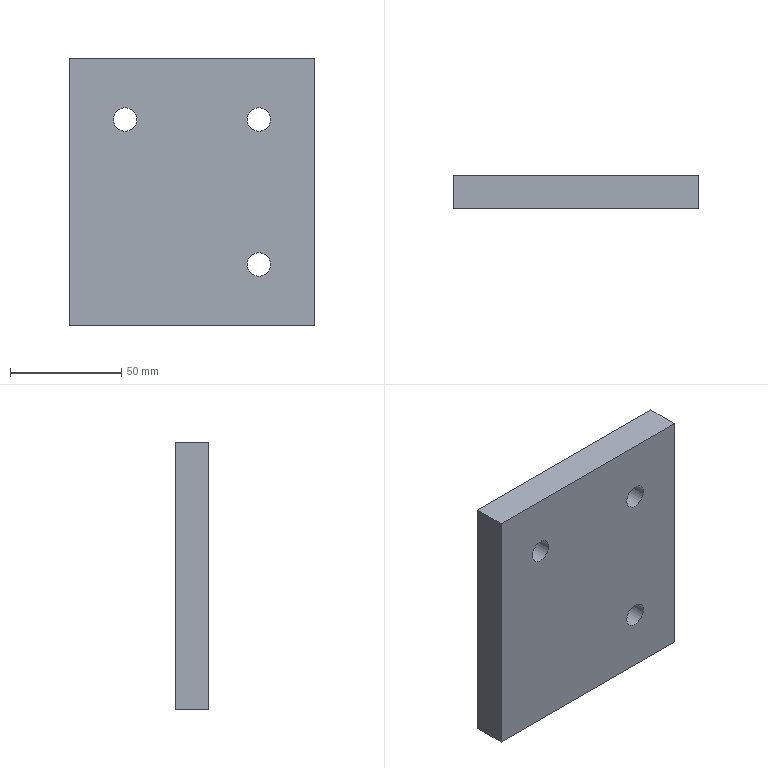Component | NX | FIXED_PLATE_2 | 1 solid | 9 faces | box 110 x 15 x 120 mm | volume 194103 mm3 | plane 6 | cylinder 3 | commonest cylinder face diameters 10.5 x3
STEP:
#1=CARTESIAN_POINT('',(0.,0.,0.));
#2=DIRECTION('',(0.,0.,1.));
#3=DIRECTION('',(1.,0.,0.));
#4=AXIS2_PLACEMENT_3D('',#1,#2,#3);
#5=CARTESIAN_POINT('',(1379.254,1145.,643.5));
#6=VERTEX_POINT('',#5);
#7=CARTESIAN_POINT('',(1379.254,1145.,763.5));
#8=VERTEX_POINT('',#7);
#9=CARTESIAN_POINT('',(1379.254,1145.,643.5));
#10=DIRECTION('',(0.,0.,1.));
#11=VECTOR('',#10,1.);
#12=LINE('',#9,#11);
#13=CARTESIAN_POINT('',(1379.254,1160.,643.5));
#14=DIRECTION('',(1.,0.,0.));
#15=DIRECTION('',(0.,0.,-1.));
#16=AXIS2_PLACEMENT_3D('',#13,#14,#15);
#17=PLANE('',#16);
#18=CARTESIAN_POINT('',(0.,-15.));
#19=DIRECTION('',(-1.,0.));
#20=VECTOR('',#19,1.);
#21=LINE('',#18,#20);
#22=(GEOMETRIC_REPRESENTATION_CONTEXT(2)PARAMETRIC_REPRESENTATION_CONTEXT()REPRESENTATION_CONTEXT('',''));
#23=DEFINITIONAL_REPRESENTATION('',(#21),#22);
#24=PCURVE('',#17,#23);
#25=CARTESIAN_POINT('',(1404.254,1145.,736.));
#26=DIRECTION('',(0.,1.,0.));
#27=DIRECTION('',(0.,0.,1.));
#28=AXIS2_PLACEMENT_3D('',#25,#26,#27);
#29=PLANE('',#28);
#30=CARTESIAN_POINT('',(-92.5,-25.));
#31=DIRECTION('',(1.,0.));
#32=VECTOR('',#31,1.);
#33=LINE('',#30,#32);
#34=(GEOMETRIC_REPRESENTATION_CONTEXT(2)PARAMETRIC_REPRESENTATION_CONTEXT()REPRESENTATION_CONTEXT('',''));
#35=DEFINITIONAL_REPRESENTATION('',(#33),#34);
#36=PCURVE('',#29,#35);
#37=SURFACE_CURVE('',#12,(#24,#36),.PCURVE_S1.);
#38=EDGE_CURVE('',#6,#8,#37,.T.);
#39=ORIENTED_EDGE('',*,*,#38,.T.);
#40=CARTESIAN_POINT('',(1379.254,1160.,763.5));
#41=VERTEX_POINT('',#40);
#42=CARTESIAN_POINT('',(1379.254,1160.,763.5));
#43=DIRECTION('',(0.,-1.,0.));
#44=VECTOR('',#43,1.);
#45=LINE('',#42,#44);
#46=CARTESIAN_POINT('',(-120.,0.));
#47=DIRECTION('',(0.,-1.));
#48=VECTOR('',#47,1.);
#49=LINE('',#46,#48);
#50=(GEOMETRIC_REPRESENTATION_CONTEXT(2)PARAMETRIC_REPRESENTATION_CONTEXT()REPRESENTATION_CONTEXT('',''));
#51=DEFINITIONAL_REPRESENTATION('',(#49),#50);
#52=PCURVE('',#17,#51);
#53=CARTESIAN_POINT('',(1379.254,1160.,763.5));
#54=DIRECTION('',(0.,0.,-1.));
#55=DIRECTION('',(-1.,0.,-0.));
#56=AXIS2_PLACEMENT_3D('',#53,#54,#55);
#57=PLANE('',#56);
#58=CARTESIAN_POINT('',(0.,0.));
#59=DIRECTION('',(0.,-1.));
#60=VECTOR('',#59,1.);
#61=LINE('',#58,#60);
#62=(GEOMETRIC_REPRESENTATION_CONTEXT(2)PARAMETRIC_REPRESENTATION_CONTEXT()REPRESENTATION_CONTEXT('',''));
#63=DEFINITIONAL_REPRESENTATION('',(#61),#62);
#64=PCURVE('',#57,#63);
#65=SURFACE_CURVE('',#45,(#52,#64),.PCURVE_S1.);
#66=EDGE_CURVE('',#41,#8,#65,.T.);
#67=ORIENTED_EDGE('',*,*,#66,.F.);
#68=CARTESIAN_POINT('',(1379.254,1160.,643.5));
#69=VERTEX_POINT('',#68);
#70=CARTESIAN_POINT('',(1379.254,1160.,643.5));
#71=DIRECTION('',(0.,0.,1.));
#72=VECTOR('',#71,1.);
#73=LINE('',#70,#72);
#74=CARTESIAN_POINT('',(0.,0.));
#75=DIRECTION('',(-1.,0.));
#76=VECTOR('',#75,1.);
#77=LINE('',#74,#76);
#78=(GEOMETRIC_REPRESENTATION_CONTEXT(2)PARAMETRIC_REPRESENTATION_CONTEXT()REPRESENTATION_CONTEXT('',''));
#79=DEFINITIONAL_REPRESENTATION('',(#77),#78);
#80=PCURVE('',#17,#79);
#81=CARTESIAN_POINT('',(1404.254,1160.,736.));
#82=DIRECTION('',(0.,1.,0.));
#83=DIRECTION('',(0.,0.,1.));
#84=AXIS2_PLACEMENT_3D('',#81,#82,#83);
#85=PLANE('',#84);
#86=CARTESIAN_POINT('',(-92.5,-25.));
#87=DIRECTION('',(1.,0.));
#88=VECTOR('',#87,1.);
#89=LINE('',#86,#88);
#90=(GEOMETRIC_REPRESENTATION_CONTEXT(2)PARAMETRIC_REPRESENTATION_CONTEXT()REPRESENTATION_CONTEXT('',''));
#91=DEFINITIONAL_REPRESENTATION('',(#89),#90);
#92=PCURVE('',#85,#91);
#93=SURFACE_CURVE('',#73,(#80,#92),.PCURVE_S1.);
#94=EDGE_CURVE('',#69,#41,#93,.T.);
#95=ORIENTED_EDGE('',*,*,#94,.F.);
#96=CARTESIAN_POINT('',(1379.254,1160.,643.5));
#97=DIRECTION('',(0.,-1.,0.));
#98=VECTOR('',#97,1.);
#99=LINE('',#96,#98);
#100=CARTESIAN_POINT('',(0.,0.));
#101=DIRECTION('',(0.,-1.));
#102=VECTOR('',#101,1.);
#103=LINE('',#100,#102);
#104=(GEOMETRIC_REPRESENTATION_CONTEXT(2)PARAMETRIC_REPRESENTATION_CONTEXT()REPRESENTATION_CONTEXT('',''));
#105=DEFINITIONAL_REPRESENTATION('',(#103),#104);
#106=PCURVE('',#17,#105);
#107=CARTESIAN_POINT('',(1489.254,1160.,643.5));
#108=DIRECTION('',(0.,0.,1.));
#109=DIRECTION('',(1.,0.,0.));
#110=AXIS2_PLACEMENT_3D('',#107,#108,#109);
#111=PLANE('',#110);
#112=CARTESIAN_POINT('',(-110.,0.));
#113=DIRECTION('',(0.,-1.));
#114=VECTOR('',#113,1.);
#115=LINE('',#112,#114);
#116=(GEOMETRIC_REPRESENTATION_CONTEXT(2)PARAMETRIC_REPRESENTATION_CONTEXT()REPRESENTATION_CONTEXT('',''));
#117=DEFINITIONAL_REPRESENTATION('',(#115),#116);
#118=PCURVE('',#111,#117);
#119=SURFACE_CURVE('',#99,(#106,#118),.PCURVE_S1.);
#120=EDGE_CURVE('',#69,#6,#119,.T.);
#121=ORIENTED_EDGE('',*,*,#120,.T.);
#122=EDGE_LOOP('',(#39,#67,#95,#121));
#123=FACE_BOUND('',#122,.T.);
#124=ADVANCED_FACE('',(#123),#17,.F.);
#125=CARTESIAN_POINT('',(1489.254,1145.,763.5));
#126=VERTEX_POINT('',#125);
#127=CARTESIAN_POINT('',(1379.254,1145.,763.5));
#128=DIRECTION('',(1.,0.,0.));
#129=VECTOR('',#128,1.);
#130=LINE('',#127,#129);
#131=CARTESIAN_POINT('',(0.,-15.));
#132=DIRECTION('',(-1.,0.));
#133=VECTOR('',#132,1.);
#134=LINE('',#131,#133);
#135=(GEOMETRIC_REPRESENTATION_CONTEXT(2)PARAMETRIC_REPRESENTATION_CONTEXT()REPRESENTATION_CONTEXT('',''));
#136=DEFINITIONAL_REPRESENTATION('',(#134),#135);
#137=PCURVE('',#57,#136);
#138=CARTESIAN_POINT('',(27.5,-25.));
#139=DIRECTION('',(0.,1.));
#140=VECTOR('',#139,1.);
#141=LINE('',#138,#140);
#142=(GEOMETRIC_REPRESENTATION_CONTEXT(2)PARAMETRIC_REPRESENTATION_CONTEXT()REPRESENTATION_CONTEXT('',''));
#143=DEFINITIONAL_REPRESENTATION('',(#141),#142);
#144=PCURVE('',#29,#143);
#145=SURFACE_CURVE('',#130,(#137,#144),.PCURVE_S1.);
#146=EDGE_CURVE('',#8,#126,#145,.T.);
#147=ORIENTED_EDGE('',*,*,#146,.T.);
#148=CARTESIAN_POINT('',(1489.254,1160.,763.5));
#149=VERTEX_POINT('',#148);
#150=CARTESIAN_POINT('',(1489.254,1160.,763.5));
#151=DIRECTION('',(0.,-1.,0.));
#152=VECTOR('',#151,1.);
#153=LINE('',#150,#152);
#154=CARTESIAN_POINT('',(-110.,0.));
#155=DIRECTION('',(0.,-1.));
#156=VECTOR('',#155,1.);
#157=LINE('',#154,#156);
#158=(GEOMETRIC_REPRESENTATION_CONTEXT(2)PARAMETRIC_REPRESENTATION_CONTEXT()REPRESENTATION_CONTEXT('',''));
#159=DEFINITIONAL_REPRESENTATION('',(#157),#158);
#160=PCURVE('',#57,#159);
#161=CARTESIAN_POINT('',(1489.254,1160.,763.5));
#162=DIRECTION('',(-1.,0.,-0.));
#163=DIRECTION('',(-0.,0.,1.));
#164=AXIS2_PLACEMENT_3D('',#161,#162,#163);
#165=PLANE('',#164);
#166=CARTESIAN_POINT('',(0.,0.));
#167=DIRECTION('',(0.,-1.));
#168=VECTOR('',#167,1.);
#169=LINE('',#166,#168);
#170=(GEOMETRIC_REPRESENTATION_CONTEXT(2)PARAMETRIC_REPRESENTATION_CONTEXT()REPRESENTATION_CONTEXT('',''));
#171=DEFINITIONAL_REPRESENTATION('',(#169),#170);
#172=PCURVE('',#165,#171);
#173=SURFACE_CURVE('',#153,(#160,#172),.PCURVE_S1.);
#174=EDGE_CURVE('',#149,#126,#173,.T.);
#175=ORIENTED_EDGE('',*,*,#174,.F.);
#176=CARTESIAN_POINT('',(1379.254,1160.,763.5));
#177=DIRECTION('',(1.,0.,0.));
#178=VECTOR('',#177,1.);
#179=LINE('',#176,#178);
#180=CARTESIAN_POINT('',(0.,0.));
#181=DIRECTION('',(-1.,0.));
#182=VECTOR('',#181,1.);
#183=LINE('',#180,#182);
#184=(GEOMETRIC_REPRESENTATION_CONTEXT(2)PARAMETRIC_REPRESENTATION_CONTEXT()REPRESENTATION_CONTEXT('',''));
#185=DEFINITIONAL_REPRESENTATION('',(#183),#184);
#186=PCURVE('',#57,#185);
#187=CARTESIAN_POINT('',(27.5,-25.));
#188=DIRECTION('',(0.,1.));
#189=VECTOR('',#188,1.);
#190=LINE('',#187,#189);
#191=(GEOMETRIC_REPRESENTATION_CONTEXT(2)PARAMETRIC_REPRESENTATION_CONTEXT()REPRESENTATION_CONTEXT('',''));
#192=DEFINITIONAL_REPRESENTATION('',(#190),#191);
#193=PCURVE('',#85,#192);
#194=SURFACE_CURVE('',#179,(#186,#193),.PCURVE_S1.);
#195=EDGE_CURVE('',#41,#149,#194,.T.);
#196=ORIENTED_EDGE('',*,*,#195,.F.);
#197=ORIENTED_EDGE('',*,*,#66,.T.);
#198=EDGE_LOOP('',(#147,#175,#196,#197));
#199=FACE_BOUND('',#198,.T.);
#200=ADVANCED_FACE('',(#199),#57,.F.);
#201=CARTESIAN_POINT('',(1489.254,1145.,643.5));
#202=VERTEX_POINT('',#201);
#203=CARTESIAN_POINT('',(1489.254,1145.,763.5));
#204=DIRECTION('',(0.,0.,-1.));
#205=VECTOR('',#204,1.);
#206=LINE('',#203,#205);
#207=CARTESIAN_POINT('',(0.,-15.));
#208=DIRECTION('',(-1.,0.));
#209=VECTOR('',#208,1.);
#210=LINE('',#207,#209);
#211=(GEOMETRIC_REPRESENTATION_CONTEXT(2)PARAMETRIC_REPRESENTATION_CONTEXT()REPRESENTATION_CONTEXT('',''));
#212=DEFINITIONAL_REPRESENTATION('',(#210),#211);
#213=PCURVE('',#165,#212);
#214=CARTESIAN_POINT('',(27.5,85.));
#215=DIRECTION('',(-1.,0.));
#216=VECTOR('',#215,1.);
#217=LINE('',#214,#216);
#218=(GEOMETRIC_REPRESENTATION_CONTEXT(2)PARAMETRIC_REPRESENTATION_CONTEXT()REPRESENTATION_CONTEXT('',''));
#219=DEFINITIONAL_REPRESENTATION('',(#217),#218);
#220=PCURVE('',#29,#219);
#221=SURFACE_CURVE('',#206,(#213,#220),.PCURVE_S1.);
#222=EDGE_CURVE('',#126,#202,#221,.T.);
#223=ORIENTED_EDGE('',*,*,#222,.T.);
#224=CARTESIAN_POINT('',(1489.254,1160.,643.5));
#225=VERTEX_POINT('',#224);
#226=CARTESIAN_POINT('',(1489.254,1160.,643.5));
#227=DIRECTION('',(0.,-1.,0.));
#228=VECTOR('',#227,1.);
#229=LINE('',#226,#228);
#230=CARTESIAN_POINT('',(-120.,0.));
#231=DIRECTION('',(0.,-1.));
#232=VECTOR('',#231,1.);
#233=LINE('',#230,#232);
#234=(GEOMETRIC_REPRESENTATION_CONTEXT(2)PARAMETRIC_REPRESENTATION_CONTEXT()REPRESENTATION_CONTEXT('',''));
#235=DEFINITIONAL_REPRESENTATION('',(#233),#234);
#236=PCURVE('',#165,#235);
#237=CARTESIAN_POINT('',(0.,0.));
#238=DIRECTION('',(0.,-1.));
#239=VECTOR('',#238,1.);
#240=LINE('',#237,#239);
#241=(GEOMETRIC_REPRESENTATION_CONTEXT(2)PARAMETRIC_REPRESENTATION_CONTEXT()REPRESENTATION_CONTEXT('',''));
#242=DEFINITIONAL_REPRESENTATION('',(#240),#241);
#243=PCURVE('',#111,#242);
#244=SURFACE_CURVE('',#229,(#236,#243),.PCURVE_S1.);
#245=EDGE_CURVE('',#225,#202,#244,.T.);
#246=ORIENTED_EDGE('',*,*,#245,.F.);
#247=CARTESIAN_POINT('',(1489.254,1160.,763.5));
#248=DIRECTION('',(0.,0.,-1.));
#249=VECTOR('',#248,1.);
#250=LINE('',#247,#249);
#251=CARTESIAN_POINT('',(0.,0.));
#252=DIRECTION('',(-1.,0.));
#253=VECTOR('',#252,1.);
#254=LINE('',#251,#253);
#255=(GEOMETRIC_REPRESENTATION_CONTEXT(2)PARAMETRIC_REPRESENTATION_CONTEXT()REPRESENTATION_CONTEXT('',''));
#256=DEFINITIONAL_REPRESENTATION('',(#254),#255);
#257=PCURVE('',#165,#256);
#258=CARTESIAN_POINT('',(27.5,85.));
#259=DIRECTION('',(-1.,0.));
#260=VECTOR('',#259,1.);
#261=LINE('',#258,#260);
#262=(GEOMETRIC_REPRESENTATION_CONTEXT(2)PARAMETRIC_REPRESENTATION_CONTEXT()REPRESENTATION_CONTEXT('',''));
#263=DEFINITIONAL_REPRESENTATION('',(#261),#262);
#264=PCURVE('',#85,#263);
#265=SURFACE_CURVE('',#250,(#257,#264),.PCURVE_S1.);
#266=EDGE_CURVE('',#149,#225,#265,.T.);
#267=ORIENTED_EDGE('',*,*,#266,.F.);
#268=ORIENTED_EDGE('',*,*,#174,.T.);
#269=EDGE_LOOP('',(#223,#246,#267,#268));
#270=FACE_BOUND('',#269,.T.);
#271=ADVANCED_FACE('',(#270),#165,.F.);
#272=CARTESIAN_POINT('',(1469.504,1160.,671.));
#273=VERTEX_POINT('',#272);
#274=CARTESIAN_POINT('',(1464.254,1160.,671.));
#275=DIRECTION('',(0.,1.,0.));
#276=DIRECTION('',(1.,0.,0.));
#277=AXIS2_PLACEMENT_3D('',#274,#275,#276);
#278=CIRCLE('',#277,5.25);
#279=CARTESIAN_POINT('',(1464.254,1160.,671.));
#280=DIRECTION('',(0.,-1.,0.));
#281=DIRECTION('',(0.,0.,-1.));
#282=AXIS2_PLACEMENT_3D('',#279,#280,#281);
#283=CYLINDRICAL_SURFACE('',#282,5.25);
#284=CARTESIAN_POINT('',(7.854,0.));
#285=DIRECTION('',(-1.,0.));
#286=VECTOR('',#285,1.);
#287=LINE('',#284,#286);
#288=(GEOMETRIC_REPRESENTATION_CONTEXT(2)PARAMETRIC_REPRESENTATION_CONTEXT()REPRESENTATION_CONTEXT('',''));
#289=DEFINITIONAL_REPRESENTATION('',(#287),#288);
#290=PCURVE('',#283,#289);
#291=CARTESIAN_POINT('',(-65.,60.));
#292=DIRECTION('',(0.,1.));
#293=AXIS2_PLACEMENT_2D('',#291,#292);
#294=CIRCLE('',#293,5.25);
#295=(GEOMETRIC_REPRESENTATION_CONTEXT(2)PARAMETRIC_REPRESENTATION_CONTEXT()REPRESENTATION_CONTEXT('',''));
#296=DEFINITIONAL_REPRESENTATION('',(#294),#295);
#297=PCURVE('',#85,#296);
#298=SURFACE_CURVE('',#278,(#290,#297),.PCURVE_S1.);
#299=EDGE_CURVE('',#273,#273,#298,.T.);
#300=ORIENTED_EDGE('',*,*,#299,.F.);
#301=CARTESIAN_POINT('',(1469.504,1145.,671.));
#302=VERTEX_POINT('',#301);
#303=CARTESIAN_POINT('',(1469.504,1160.,671.));
#304=CARTESIAN_POINT('',(1469.504,1145.,671.));
#305=B_SPLINE_CURVE_WITH_KNOTS('',1,(#303,#304),.UNSPECIFIED.,.F.,.F.,(2,2),(0.,15.),.PIECEWISE_BEZIER_KNOTS.);
#306=CARTESIAN_POINT('',(7.854,0.));
#307=DIRECTION('',(0.,1.));
#308=VECTOR('',#307,1.);
#309=LINE('',#306,#308);
#310=(GEOMETRIC_REPRESENTATION_CONTEXT(2)PARAMETRIC_REPRESENTATION_CONTEXT()REPRESENTATION_CONTEXT('',''));
#311=DEFINITIONAL_REPRESENTATION('',(#309),#310);
#312=PCURVE('',#283,#311);
#313=CARTESIAN_POINT('',(1.571,0.));
#314=DIRECTION('',(0.,1.));
#315=VECTOR('',#314,1.);
#316=LINE('',#313,#315);
#317=(GEOMETRIC_REPRESENTATION_CONTEXT(2)PARAMETRIC_REPRESENTATION_CONTEXT()REPRESENTATION_CONTEXT('',''));
#318=DEFINITIONAL_REPRESENTATION('',(#316),#317);
#319=PCURVE('',#283,#318);
#320=SEAM_CURVE('',#305,(#312,#319),.PCURVE_S1.);
#321=EDGE_CURVE('',#273,#302,#320,.T.);
#322=ORIENTED_EDGE('',*,*,#321,.T.);
#323=CARTESIAN_POINT('',(1464.254,1145.,671.));
#324=DIRECTION('',(0.,1.,0.));
#325=DIRECTION('',(1.,0.,0.));
#326=AXIS2_PLACEMENT_3D('',#323,#324,#325);
#327=CIRCLE('',#326,5.25);
#328=CARTESIAN_POINT('',(7.854,15.));
#329=DIRECTION('',(-1.,0.));
#330=VECTOR('',#329,1.);
#331=LINE('',#328,#330);
#332=(GEOMETRIC_REPRESENTATION_CONTEXT(2)PARAMETRIC_REPRESENTATION_CONTEXT()REPRESENTATION_CONTEXT('',''));
#333=DEFINITIONAL_REPRESENTATION('',(#331),#332);
#334=PCURVE('',#283,#333);
#335=CARTESIAN_POINT('',(-65.,60.));
#336=DIRECTION('',(0.,1.));
#337=AXIS2_PLACEMENT_2D('',#335,#336);
#338=CIRCLE('',#337,5.25);
#339=(GEOMETRIC_REPRESENTATION_CONTEXT(2)PARAMETRIC_REPRESENTATION_CONTEXT()REPRESENTATION_CONTEXT('',''));
#340=DEFINITIONAL_REPRESENTATION('',(#338),#339);
#341=PCURVE('',#29,#340);
#342=SURFACE_CURVE('',#327,(#334,#341),.PCURVE_S1.);
#343=EDGE_CURVE('',#302,#302,#342,.T.);
#344=ORIENTED_EDGE('',*,*,#343,.T.);
#345=ORIENTED_EDGE('',*,*,#321,.F.);
#346=EDGE_LOOP('',(#300,#322,#344,#345));
#347=FACE_BOUND('',#346,.F.);
#348=ADVANCED_FACE('',(#347),#283,.F.);
#349=CARTESIAN_POINT('',(1409.504,1160.,736.));
#350=VERTEX_POINT('',#349);
#351=CARTESIAN_POINT('',(1404.254,1160.,736.));
#352=DIRECTION('',(0.,1.,0.));
#353=DIRECTION('',(1.,0.,0.));
#354=AXIS2_PLACEMENT_3D('',#351,#352,#353);
#355=CIRCLE('',#354,5.25);
#356=CARTESIAN_POINT('',(1404.254,1160.,736.));
#357=DIRECTION('',(0.,-1.,0.));
#358=DIRECTION('',(0.,0.,-1.));
#359=AXIS2_PLACEMENT_3D('',#356,#357,#358);
#360=CYLINDRICAL_SURFACE('',#359,5.25);
#361=CARTESIAN_POINT('',(7.854,0.));
#362=DIRECTION('',(-1.,0.));
#363=VECTOR('',#362,1.);
#364=LINE('',#361,#363);
#365=(GEOMETRIC_REPRESENTATION_CONTEXT(2)PARAMETRIC_REPRESENTATION_CONTEXT()REPRESENTATION_CONTEXT('',''));
#366=DEFINITIONAL_REPRESENTATION('',(#364),#365);
#367=PCURVE('',#360,#366);
#368=CARTESIAN_POINT('',(0.,0.));
#369=DIRECTION('',(0.,1.));
#370=AXIS2_PLACEMENT_2D('',#368,#369);
#371=CIRCLE('',#370,5.25);
#372=(GEOMETRIC_REPRESENTATION_CONTEXT(2)PARAMETRIC_REPRESENTATION_CONTEXT()REPRESENTATION_CONTEXT('',''));
#373=DEFINITIONAL_REPRESENTATION('',(#371),#372);
#374=PCURVE('',#85,#373);
#375=SURFACE_CURVE('',#355,(#367,#374),.PCURVE_S1.);
#376=EDGE_CURVE('',#350,#350,#375,.T.);
#377=ORIENTED_EDGE('',*,*,#376,.F.);
#378=CARTESIAN_POINT('',(1409.504,1145.,736.));
#379=VERTEX_POINT('',#378);
#380=CARTESIAN_POINT('',(1409.504,1160.,736.));
#381=CARTESIAN_POINT('',(1409.504,1145.,736.));
#382=B_SPLINE_CURVE_WITH_KNOTS('',1,(#380,#381),.UNSPECIFIED.,.F.,.F.,(2,2),(0.,15.),.PIECEWISE_BEZIER_KNOTS.);
#383=CARTESIAN_POINT('',(7.854,0.));
#384=DIRECTION('',(0.,1.));
#385=VECTOR('',#384,1.);
#386=LINE('',#383,#385);
#387=(GEOMETRIC_REPRESENTATION_CONTEXT(2)PARAMETRIC_REPRESENTATION_CONTEXT()REPRESENTATION_CONTEXT('',''));
#388=DEFINITIONAL_REPRESENTATION('',(#386),#387);
#389=PCURVE('',#360,#388);
#390=CARTESIAN_POINT('',(1.571,0.));
#391=DIRECTION('',(0.,1.));
#392=VECTOR('',#391,1.);
#393=LINE('',#390,#392);
#394=(GEOMETRIC_REPRESENTATION_CONTEXT(2)PARAMETRIC_REPRESENTATION_CONTEXT()REPRESENTATION_CONTEXT('',''));
#395=DEFINITIONAL_REPRESENTATION('',(#393),#394);
#396=PCURVE('',#360,#395);
#397=SEAM_CURVE('',#382,(#389,#396),.PCURVE_S1.);
#398=EDGE_CURVE('',#350,#379,#397,.T.);
#399=ORIENTED_EDGE('',*,*,#398,.T.);
#400=CARTESIAN_POINT('',(1404.254,1145.,736.));
#401=DIRECTION('',(0.,1.,0.));
#402=DIRECTION('',(1.,0.,0.));
#403=AXIS2_PLACEMENT_3D('',#400,#401,#402);
#404=CIRCLE('',#403,5.25);
#405=CARTESIAN_POINT('',(7.854,15.));
#406=DIRECTION('',(-1.,0.));
#407=VECTOR('',#406,1.);
#408=LINE('',#405,#407);
#409=(GEOMETRIC_REPRESENTATION_CONTEXT(2)PARAMETRIC_REPRESENTATION_CONTEXT()REPRESENTATION_CONTEXT('',''));
#410=DEFINITIONAL_REPRESENTATION('',(#408),#409);
#411=PCURVE('',#360,#410);
#412=CARTESIAN_POINT('',(0.,0.));
#413=DIRECTION('',(0.,1.));
#414=AXIS2_PLACEMENT_2D('',#412,#413);
#415=CIRCLE('',#414,5.25);
#416=(GEOMETRIC_REPRESENTATION_CONTEXT(2)PARAMETRIC_REPRESENTATION_CONTEXT()REPRESENTATION_CONTEXT('',''));
#417=DEFINITIONAL_REPRESENTATION('',(#415),#416);
#418=PCURVE('',#29,#417);
#419=SURFACE_CURVE('',#404,(#411,#418),.PCURVE_S1.);
#420=EDGE_CURVE('',#379,#379,#419,.T.);
#421=ORIENTED_EDGE('',*,*,#420,.T.);
#422=ORIENTED_EDGE('',*,*,#398,.F.);
#423=EDGE_LOOP('',(#377,#399,#421,#422));
#424=FACE_BOUND('',#423,.F.);
#425=ADVANCED_FACE('',(#424),#360,.F.);
#426=CARTESIAN_POINT('',(1489.254,1145.,643.5));
#427=DIRECTION('',(-1.,0.,0.));
#428=VECTOR('',#427,1.);
#429=LINE('',#426,#428);
#430=CARTESIAN_POINT('',(0.,-15.));
#431=DIRECTION('',(-1.,0.));
#432=VECTOR('',#431,1.);
#433=LINE('',#430,#432);
#434=(GEOMETRIC_REPRESENTATION_CONTEXT(2)PARAMETRIC_REPRESENTATION_CONTEXT()REPRESENTATION_CONTEXT('',''));
#435=DEFINITIONAL_REPRESENTATION('',(#433),#434);
#436=PCURVE('',#111,#435);
#437=CARTESIAN_POINT('',(-92.5,85.));
#438=DIRECTION('',(0.,-1.));
#439=VECTOR('',#438,1.);
#440=LINE('',#437,#439);
#441=(GEOMETRIC_REPRESENTATION_CONTEXT(2)PARAMETRIC_REPRESENTATION_CONTEXT()REPRESENTATION_CONTEXT('',''));
#442=DEFINITIONAL_REPRESENTATION('',(#440),#441);
#443=PCURVE('',#29,#442);
#444=SURFACE_CURVE('',#429,(#436,#443),.PCURVE_S1.);
#445=EDGE_CURVE('',#202,#6,#444,.T.);
#446=ORIENTED_EDGE('',*,*,#445,.T.);
#447=ORIENTED_EDGE('',*,*,#120,.F.);
#448=CARTESIAN_POINT('',(1489.254,1160.,643.5));
#449=DIRECTION('',(-1.,0.,0.));
#450=VECTOR('',#449,1.);
#451=LINE('',#448,#450);
#452=CARTESIAN_POINT('',(0.,0.));
#453=DIRECTION('',(-1.,0.));
#454=VECTOR('',#453,1.);
#455=LINE('',#452,#454);
#456=(GEOMETRIC_REPRESENTATION_CONTEXT(2)PARAMETRIC_REPRESENTATION_CONTEXT()REPRESENTATION_CONTEXT('',''));
#457=DEFINITIONAL_REPRESENTATION('',(#455),#456);
#458=PCURVE('',#111,#457);
#459=CARTESIAN_POINT('',(-92.5,85.));
#460=DIRECTION('',(0.,-1.));
#461=VECTOR('',#460,1.);
#462=LINE('',#459,#461);
#463=(GEOMETRIC_REPRESENTATION_CONTEXT(2)PARAMETRIC_REPRESENTATION_CONTEXT()REPRESENTATION_CONTEXT('',''));
#464=DEFINITIONAL_REPRESENTATION('',(#462),#463);
#465=PCURVE('',#85,#464);
#466=SURFACE_CURVE('',#451,(#458,#465),.PCURVE_S1.);
#467=EDGE_CURVE('',#225,#69,#466,.T.);
#468=ORIENTED_EDGE('',*,*,#467,.F.);
#469=ORIENTED_EDGE('',*,*,#245,.T.);
#470=EDGE_LOOP('',(#446,#447,#468,#469));
#471=FACE_BOUND('',#470,.T.);
#472=ADVANCED_FACE('',(#471),#111,.F.);
#473=CARTESIAN_POINT('',(1469.504,1160.,736.));
#474=VERTEX_POINT('',#473);
#475=CARTESIAN_POINT('',(1464.254,1160.,736.));
#476=DIRECTION('',(0.,1.,0.));
#477=DIRECTION('',(1.,0.,0.));
#478=AXIS2_PLACEMENT_3D('',#475,#476,#477);
#479=CIRCLE('',#478,5.25);
#480=CARTESIAN_POINT('',(1464.254,1160.,736.));
#481=DIRECTION('',(0.,-1.,0.));
#482=DIRECTION('',(0.,0.,-1.));
#483=AXIS2_PLACEMENT_3D('',#480,#481,#482);
#484=CYLINDRICAL_SURFACE('',#483,5.25);
#485=CARTESIAN_POINT('',(7.854,0.));
#486=DIRECTION('',(-1.,0.));
#487=VECTOR('',#486,1.);
#488=LINE('',#485,#487);
#489=(GEOMETRIC_REPRESENTATION_CONTEXT(2)PARAMETRIC_REPRESENTATION_CONTEXT()REPRESENTATION_CONTEXT('',''));
#490=DEFINITIONAL_REPRESENTATION('',(#488),#489);
#491=PCURVE('',#484,#490);
#492=CARTESIAN_POINT('',(0.,60.));
#493=DIRECTION('',(0.,1.));
#494=AXIS2_PLACEMENT_2D('',#492,#493);
#495=CIRCLE('',#494,5.25);
#496=(GEOMETRIC_REPRESENTATION_CONTEXT(2)PARAMETRIC_REPRESENTATION_CONTEXT()REPRESENTATION_CONTEXT('',''));
#497=DEFINITIONAL_REPRESENTATION('',(#495),#496);
#498=PCURVE('',#85,#497);
#499=SURFACE_CURVE('',#479,(#491,#498),.PCURVE_S1.);
#500=EDGE_CURVE('',#474,#474,#499,.T.);
#501=ORIENTED_EDGE('',*,*,#500,.F.);
#502=CARTESIAN_POINT('',(1469.504,1145.,736.));
#503=VERTEX_POINT('',#502);
#504=CARTESIAN_POINT('',(1469.504,1160.,736.));
#505=CARTESIAN_POINT('',(1469.504,1145.,736.));
#506=B_SPLINE_CURVE_WITH_KNOTS('',1,(#504,#505),.UNSPECIFIED.,.F.,.F.,(2,2),(0.,15.),.PIECEWISE_BEZIER_KNOTS.);
#507=CARTESIAN_POINT('',(7.854,0.));
#508=DIRECTION('',(0.,1.));
#509=VECTOR('',#508,1.);
#510=LINE('',#507,#509);
#511=(GEOMETRIC_REPRESENTATION_CONTEXT(2)PARAMETRIC_REPRESENTATION_CONTEXT()REPRESENTATION_CONTEXT('',''));
#512=DEFINITIONAL_REPRESENTATION('',(#510),#511);
#513=PCURVE('',#484,#512);
#514=CARTESIAN_POINT('',(1.571,0.));
#515=DIRECTION('',(0.,1.));
#516=VECTOR('',#515,1.);
#517=LINE('',#514,#516);
#518=(GEOMETRIC_REPRESENTATION_CONTEXT(2)PARAMETRIC_REPRESENTATION_CONTEXT()REPRESENTATION_CONTEXT('',''));
#519=DEFINITIONAL_REPRESENTATION('',(#517),#518);
#520=PCURVE('',#484,#519);
#521=SEAM_CURVE('',#506,(#513,#520),.PCURVE_S1.);
#522=EDGE_CURVE('',#474,#503,#521,.T.);
#523=ORIENTED_EDGE('',*,*,#522,.T.);
#524=CARTESIAN_POINT('',(1464.254,1145.,736.));
#525=DIRECTION('',(0.,1.,0.));
#526=DIRECTION('',(1.,0.,0.));
#527=AXIS2_PLACEMENT_3D('',#524,#525,#526);
#528=CIRCLE('',#527,5.25);
#529=CARTESIAN_POINT('',(7.854,15.));
#530=DIRECTION('',(-1.,0.));
#531=VECTOR('',#530,1.);
#532=LINE('',#529,#531);
#533=(GEOMETRIC_REPRESENTATION_CONTEXT(2)PARAMETRIC_REPRESENTATION_CONTEXT()REPRESENTATION_CONTEXT('',''));
#534=DEFINITIONAL_REPRESENTATION('',(#532),#533);
#535=PCURVE('',#484,#534);
#536=CARTESIAN_POINT('',(0.,60.));
#537=DIRECTION('',(0.,1.));
#538=AXIS2_PLACEMENT_2D('',#536,#537);
#539=CIRCLE('',#538,5.25);
#540=(GEOMETRIC_REPRESENTATION_CONTEXT(2)PARAMETRIC_REPRESENTATION_CONTEXT()REPRESENTATION_CONTEXT('',''));
#541=DEFINITIONAL_REPRESENTATION('',(#539),#540);
#542=PCURVE('',#29,#541);
#543=SURFACE_CURVE('',#528,(#535,#542),.PCURVE_S1.);
#544=EDGE_CURVE('',#503,#503,#543,.T.);
#545=ORIENTED_EDGE('',*,*,#544,.T.);
#546=ORIENTED_EDGE('',*,*,#522,.F.);
#547=EDGE_LOOP('',(#501,#523,#545,#546));
#548=FACE_BOUND('',#547,.F.);
#549=ADVANCED_FACE('',(#548),#484,.F.);
#550=ORIENTED_EDGE('',*,*,#94,.T.);
#551=ORIENTED_EDGE('',*,*,#195,.T.);
#552=ORIENTED_EDGE('',*,*,#266,.T.);
#553=ORIENTED_EDGE('',*,*,#467,.T.);
#554=EDGE_LOOP('',(#550,#551,#552,#553));
#555=FACE_BOUND('',#554,.T.);
#556=ORIENTED_EDGE('',*,*,#376,.F.);
#557=EDGE_LOOP('',(#556));
#558=FACE_BOUND('',#557,.T.);
#559=ORIENTED_EDGE('',*,*,#299,.F.);
#560=EDGE_LOOP('',(#559));
#561=FACE_BOUND('',#560,.T.);
#562=ORIENTED_EDGE('',*,*,#500,.F.);
#563=EDGE_LOOP('',(#562));
#564=FACE_BOUND('',#563,.T.);
#565=ADVANCED_FACE('',(#555,#558,#561,#564),#85,.T.);
#566=ORIENTED_EDGE('',*,*,#38,.F.);
#567=ORIENTED_EDGE('',*,*,#445,.F.);
#568=ORIENTED_EDGE('',*,*,#222,.F.);
#569=ORIENTED_EDGE('',*,*,#146,.F.);
#570=EDGE_LOOP('',(#566,#567,#568,#569));
#571=FACE_BOUND('',#570,.T.);
#572=ORIENTED_EDGE('',*,*,#420,.T.);
#573=EDGE_LOOP('',(#572));
#574=FACE_BOUND('',#573,.T.);
#575=ORIENTED_EDGE('',*,*,#343,.T.);
#576=EDGE_LOOP('',(#575));
#577=FACE_BOUND('',#576,.T.);
#578=ORIENTED_EDGE('',*,*,#544,.T.);
#579=EDGE_LOOP('',(#578));
#580=FACE_BOUND('',#579,.T.);
#581=ADVANCED_FACE('',(#571,#574,#577,#580),#29,.F.);
#582=CLOSED_SHELL('',(#124,#200,#271,#348,#425,#472,#549,#565,#581));
#583=MANIFOLD_SOLID_BREP('',#582);
#584=(LENGTH_UNIT()NAMED_UNIT(*)SI_UNIT(.MILLI.,.METRE.));
#585=UNCERTAINTY_MEASURE_WITH_UNIT(LENGTH_MEASURE(0.000002),#584,'','');
#586=(NAMED_UNIT(*)PLANE_ANGLE_UNIT()SI_UNIT($,.RADIAN.));
#587=(NAMED_UNIT(*)SI_UNIT($,.STERADIAN.)SOLID_ANGLE_UNIT());
#588=(GEOMETRIC_REPRESENTATION_CONTEXT(3)GLOBAL_UNCERTAINTY_ASSIGNED_CONTEXT((#585))GLOBAL_UNIT_ASSIGNED_CONTEXT((#584,#586,#587))REPRESENTATION_CONTEXT('',''));
#589=ADVANCED_BREP_SHAPE_REPRESENTATION('',(#4,#583),#588);